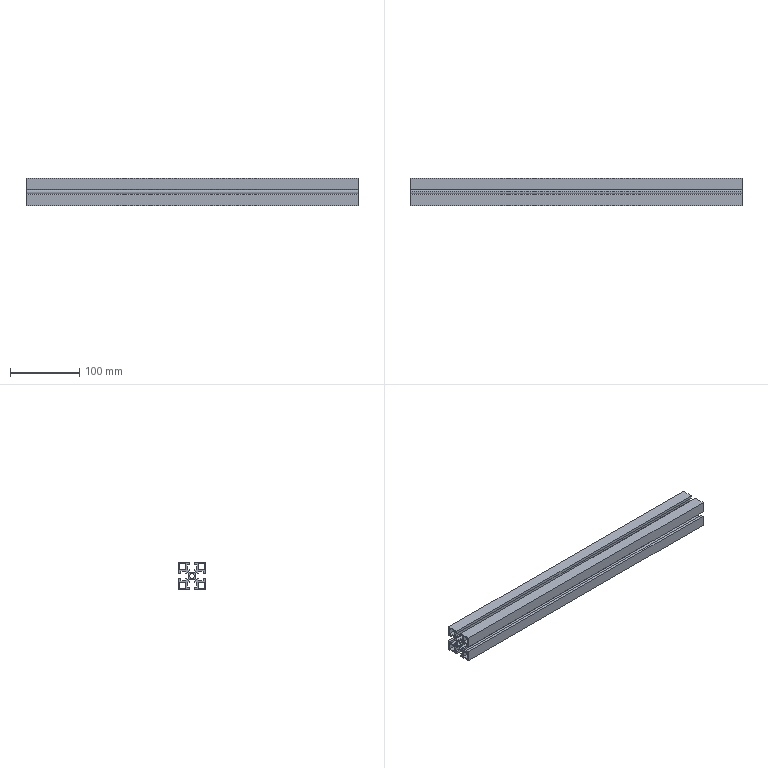Component | SolidWorks | AluminumProfile480-1 | 1 solid | 89 faces | box 480 x 40 x 40 mm | volume 278436 mm3 | plane 82 | cylinder 7 | commonest cylinder face diameters 10.5 x5 6.8 x2 | material 6061 Alloy
build123d program:
from build123d import *

# Parameters (mm, degrees)
SKETCH1_W                  = 40
SKETCH1_H                  = 40
EXTRUDE1_DEPTH             = 1640
CUT_EXTRUDE1_DEPTH         = 1641.975
SKETCH3_R                  = 3.4
CUT_EXTRUDE2_DEPTH         = 1641.975
CIRPATTERN1_COUNT          = 4
EXTRUDE2_DEPTH             = 1641.975
CIRPATTERN2_COUNT          = 4
SKETCH5_W                  = 9
SKETCH5_H                  = 9
EXTRUDE3_DEPTH             = 1641.975
CIRPATTERN3_COUNT          = 4
M8X1_25_TAPPED_HOLE3_D     = 6.8
M8X1_25_TAPPED_HOLE3_DEPTH = 19.75
M8X1_25_TAPPED_HOLE3_TIP   = 2.043
SKETCH9_W                  = 177.591
SKETCH9_H                  = 2021.808
CUT_EXTRUDE3_DEPTH         = 1641.975


with BuildPart() as part:
    # Sketch1 → Extrude1 (new body)
    with BuildSketch(Plane.XY):
        with Locations((20, 20)):
            Rectangle(SKETCH1_W, SKETCH1_H)
    extrude(amount=EXTRUDE1_DEPTH)

    # Sketch2 → Cut-Extrude1 (cut, through all)
    with BuildSketch(Plane.XY.offset(1640)):
        Polygon((16, 40), (16, 36), (13, 36), (13, 29), (27, 29), (27, 36), (24, 36), (24, 40), align=None)
    cut_extrude1 = extrude(amount=-CUT_EXTRUDE1_DEPTH, mode=Mode.SUBTRACT)

    # Sketch3 → Cut-Extrude2 (cut, through all)
    with BuildSketch(Plane.XY.offset(1640)):
        with Locations((20, 20)):
            Circle(SKETCH3_R)
    extrude(amount=-CUT_EXTRUDE2_DEPTH, mode=Mode.SUBTRACT)

    # CirPattern1: Cut-Extrude1 ×4 about axis
    cirpattern1_axis = Axis((20, 20, 0), (0, 0, 1))
    for i in range(1, CIRPATTERN1_COUNT):
        add(cut_extrude1.rotate(cirpattern1_axis, i * 360 / CIRPATTERN1_COUNT), mode=Mode.SUBTRACT)

    # Sketch4 → Extrude2 (cut, through all)
    with BuildSketch(Plane.XY.offset(1640)):
        with BuildLine():
            Line((15.75, 29), (16.457, 28.293))
            Line((16.457, 28.293), (14.806, 26.641))
            Line((14.806, 26.641), (17.082, 24.365))
            ThreePointArc((17.082, 24.365), (20, 25.25), (22.918, 24.365))
            Line((22.918, 24.365), (25.194, 26.641))
            Line((25.194, 26.641), (23.543, 28.293))
            Line((23.543, 28.293), (24.25, 29))
            Line((24.25, 29), (15.75, 29))
        make_face()
    extrude2 = extrude(amount=-EXTRUDE2_DEPTH, mode=Mode.SUBTRACT)

    # CirPattern2: Extrude2 ×4 about axis
    cirpattern2_axis = Axis((20, 20, 0), (0, 0, 1))
    for i in range(1, CIRPATTERN2_COUNT):
        add(extrude2.rotate(cirpattern2_axis, i * 360 / CIRPATTERN2_COUNT), mode=Mode.SUBTRACT)

    # Sketch5 → Extrude3 (cut, through all)
    with BuildSketch(Plane.XY.offset(1640)):
        with Locations((6.5, 33.5)):
            Rectangle(SKETCH5_W, SKETCH5_H)
    extrude3 = extrude(amount=-EXTRUDE3_DEPTH, mode=Mode.SUBTRACT)

    # CirPattern3: Extrude3 ×4 about axis
    cirpattern3_axis = Axis((20, 20, 0), (0, 0, 1))
    for i in range(1, CIRPATTERN3_COUNT):
        add(extrude3.rotate(cirpattern3_axis, i * 360 / CIRPATTERN3_COUNT), mode=Mode.SUBTRACT)

    # M8x1.25 Tapped Hole3
    with Locations(Plane(origin=(20, 20, 1640), x_dir=(1, 0, 0), z_dir=(0, 0, 1))):
        with Locations((0, 0)):
            Hole(M8X1_25_TAPPED_HOLE3_D / 2, depth=M8X1_25_TAPPED_HOLE3_DEPTH)
            with Locations((0, 0, -(M8X1_25_TAPPED_HOLE3_DEPTH + M8X1_25_TAPPED_HOLE3_TIP / 2))):  # 118° drill point
                Cone(0, M8X1_25_TAPPED_HOLE3_D / 2, M8X1_25_TAPPED_HOLE3_TIP, mode=Mode.SUBTRACT)

    # Sketch9 → Cut-Extrude3 (cut, through all)
    with BuildSketch(Plane.XZ):
        with Locations((13.869, 1490.904)):
            Rectangle(SKETCH9_W, SKETCH9_H)
    extrude(amount=-CUT_EXTRUDE3_DEPTH, mode=Mode.SUBTRACT)


solid = part.part

# Placed as in the assembly
solid = solid.moved(Location((-1248.352, -508.217, -56.285), (0, 90, 0)))